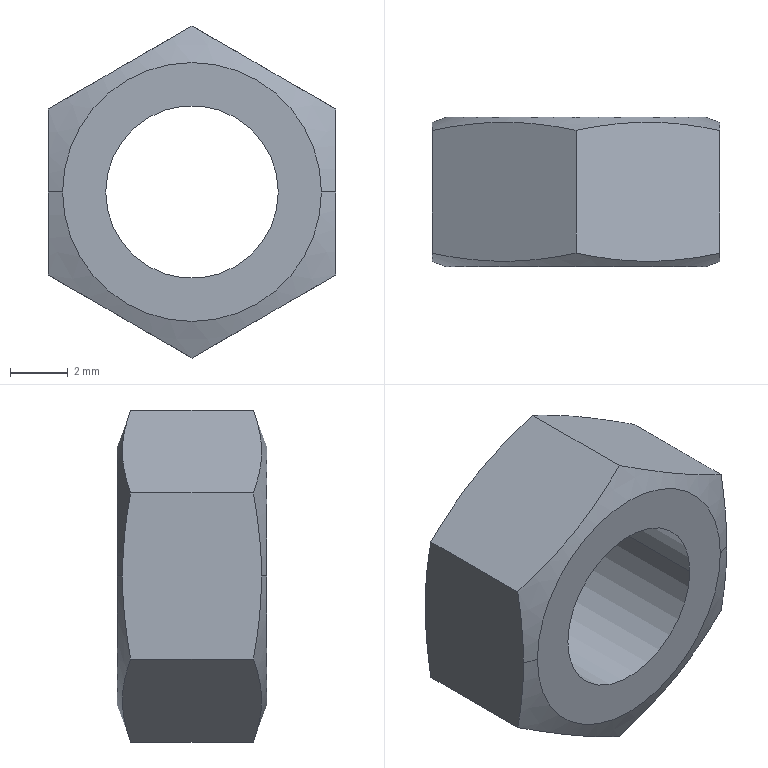Component | SolidWorks | HexNutM6-2 | 1 solid | 14 faces | box 10 x 5.2 x 11.55 mm | volume 296 mm3 | plane 8 | cone 4 | cylinder 2 | commonest cylinder face diameters 6 x2
build123d program:
from build123d import *

# Parameters (mm, degrees)
BOSS_EXTRUDE1_DEPTH = 5.2
SKETCH5_R           = 3
CUT_EXTRUDE1_DEPTH  = 10.24


with BuildPart() as part:
    # Sketch1 → Boss-Extrude1 (new body)
    with BuildSketch(Plane.XY):
        Polygon((0, 5.774), (-5, 2.887), (-5, -2.887), (0, -5.774), (5, -2.887), (5, 2.887), align=None)
    extrude(amount=BOSS_EXTRUDE1_DEPTH)

    # Sketch4 → Cut-Revolve1 (revolve, cut)
    with BuildSketch(Plane(origin=(0, 0, 0), x_dir=(0, 0, -1), z_dir=(1, 0, 0)), mode=Mode.PRIVATE) as cut_revolve1_sk:
        Polygon((-5.2, -4.5), (-4.736, -5.774), (-5.2, -5.774), align=None)
    cut_revolve1 = revolve(cut_revolve1_sk.sketch.rotate(Axis((0, 0, 5.2), (0, 0, -1)), 120), axis=Axis((0, 0, 5.2), (0, 0, -1)), mode=Mode.SUBTRACT)

    # Mirror1: Cut-Revolve1 across plane
    add(cut_revolve1.mirror(Plane.XY.offset(2.6)), mode=Mode.SUBTRACT)

    # Sketch5 → Cut-Extrude1 (cut, through all)
    with BuildSketch(Plane.XY.offset(5.2)):
        Circle(SKETCH5_R)
    extrude(amount=-CUT_EXTRUDE1_DEPTH, mode=Mode.SUBTRACT)


solid = part.part

# Placed as in the assembly
solid = solid.moved(Location((-174.718, -36.4, 23), (90, 0, 0)))
STEP:
#1=CARTESIAN_POINT('',(-6.997,-1.433,0.9055));
#2=VERTEX_POINT('',#1);
#3=CARTESIAN_POINT('',(-6.761,-1.433,0.9055));
#4=VERTEX_POINT('',#3);
#5=CARTESIAN_POINT('',(-6.879,-1.433,0.9055));
#6=DIRECTION('',(0.,-1.,0.));
#7=DIRECTION('',(1.,0.,0.));
#8=AXIS2_PLACEMENT_3D('',#5,#6,#7);
#9=CIRCLE('',#8,0.1181);
#10=EDGE_CURVE('',#2,#4,#9,.T.);
#11=ORIENTED_EDGE('',*,*,#10,.F.);
#12=CARTESIAN_POINT('',(-6.997,-1.638,0.9055));
#13=VERTEX_POINT('',#12);
#14=CARTESIAN_POINT('',(-6.997,-1.433,0.9055));
#15=DIRECTION('',(0.,-1.,0.));
#16=VECTOR('',#15,39.37);
#17=LINE('',#14,#16);
#18=EDGE_CURVE('',#2,#13,#17,.T.);
#19=ORIENTED_EDGE('',*,*,#18,.T.);
#20=CARTESIAN_POINT('',(-6.761,-1.638,0.9055));
#21=VERTEX_POINT('',#20);
#22=CARTESIAN_POINT('',(-6.879,-1.638,0.9055));
#23=DIRECTION('',(0.,-1.,0.));
#24=DIRECTION('',(1.,0.,0.));
#25=AXIS2_PLACEMENT_3D('',#22,#23,#24);
#26=CIRCLE('',#25,0.1181);
#27=EDGE_CURVE('',#13,#21,#26,.T.);
#28=ORIENTED_EDGE('',*,*,#27,.T.);
#29=CARTESIAN_POINT('',(-6.761,-1.433,0.9055));
#30=DIRECTION('',(0.,-1.,0.));
#31=VECTOR('',#30,39.37);
#32=LINE('',#29,#31);
#33=EDGE_CURVE('',#4,#21,#32,.T.);
#34=ORIENTED_EDGE('',*,*,#33,.F.);
#35=EDGE_LOOP('',(#11,#19,#28,#34));
#36=FACE_OUTER_BOUND('',#35,.T.);
#37=CARTESIAN_POINT('',(-6.879,-1.433,0.9055));
#38=DIRECTION('',(0.,-1.,0.));
#39=DIRECTION('',(1.,0.,0.));
#40=AXIS2_PLACEMENT_3D('',#37,#38,#39);
#41=CYLINDRICAL_SURFACE('',#40,0.1181);
#42=ADVANCED_FACE('',(#36),#41,.F.);
#43=CARTESIAN_POINT('',(-7.056,-1.433,0.9055));
#44=VERTEX_POINT('',#43);
#45=CARTESIAN_POINT('',(-6.702,-1.433,0.9055));
#46=VERTEX_POINT('',#45);
#47=CARTESIAN_POINT('',(-6.879,-1.433,0.9055));
#48=DIRECTION('',(0.,-1.,0.));
#49=DIRECTION('',(1.,0.,0.));
#50=AXIS2_PLACEMENT_3D('',#47,#48,#49);
#51=CIRCLE('',#50,0.1772);
#52=EDGE_CURVE('',#44,#46,#51,.T.);
#53=ORIENTED_EDGE('',*,*,#52,.T.);
#54=CARTESIAN_POINT('',(-6.682,-1.44,0.9055));
#55=VERTEX_POINT('',#54);
#56=CARTESIAN_POINT('',(-6.651,-1.451,0.9055));
#57=DIRECTION('',(0.9397,-0.342,-0.));
#58=VECTOR('',#57,39.37);
#59=LINE('',#56,#58);
#60=EDGE_CURVE('',#46,#55,#59,.T.);
#61=ORIENTED_EDGE('',*,*,#60,.T.);
#62=CARTESIAN_POINT('',(-6.682,-1.451,0.7919));
#63=VERTEX_POINT('',#62);
#64=CARTESIAN_POINT('',(-6.682,-1.451,0.7919));
#65=CARTESIAN_POINT('',(-6.682,-1.448,0.8107));
#66=CARTESIAN_POINT('',(-6.682,-1.445,0.8297));
#67=CARTESIAN_POINT('',(-6.682,-1.441,0.8676));
#68=CARTESIAN_POINT('',(-6.682,-1.44,0.8866));
#69=CARTESIAN_POINT('',(-6.682,-1.44,0.9055));
#70=B_SPLINE_CURVE_WITH_KNOTS('',3,(#64,#65,#66,#67,#68,#69),.UNSPECIFIED.,.F.,.F.,(4,2,4),(0.004893,0.006347,0.007802),.UNSPECIFIED.);
#71=EDGE_CURVE('',#63,#55,#70,.T.);
#72=ORIENTED_EDGE('',*,*,#71,.F.);
#73=CARTESIAN_POINT('',(-6.879,-1.451,0.6782));
#74=VERTEX_POINT('',#73);
#75=CARTESIAN_POINT('',(-6.879,-1.451,0.6782));
#76=CARTESIAN_POINT('',(-6.846,-1.444,0.6972));
#77=CARTESIAN_POINT('',(-6.78,-1.436,0.735));
#78=CARTESIAN_POINT('',(-6.715,-1.444,0.7729));
#79=CARTESIAN_POINT('',(-6.682,-1.451,0.7919));
#80=B_SPLINE_CURVE_WITH_KNOTS('',3,(#75,#76,#77,#78,#79),.UNSPECIFIED.,.F.,.F.,(4,1,4),(0.00000023,0.002887,0.005774),.UNSPECIFIED.);
#81=EDGE_CURVE('',#74,#63,#80,.T.);
#82=ORIENTED_EDGE('',*,*,#81,.F.);
#83=CARTESIAN_POINT('',(-7.076,-1.451,0.7919));
#84=VERTEX_POINT('',#83);
#85=CARTESIAN_POINT('',(-7.076,-1.451,0.7919));
#86=CARTESIAN_POINT('',(-7.043,-1.444,0.7729));
#87=CARTESIAN_POINT('',(-6.977,-1.436,0.735));
#88=CARTESIAN_POINT('',(-6.911,-1.444,0.6972));
#89=CARTESIAN_POINT('',(-6.879,-1.451,0.6782));
#90=B_SPLINE_CURVE_WITH_KNOTS('',3,(#85,#86,#87,#88,#89),.UNSPECIFIED.,.F.,.F.,(4,1,4),(0.00000023,0.002887,0.005774),.UNSPECIFIED.);
#91=EDGE_CURVE('',#84,#74,#90,.T.);
#92=ORIENTED_EDGE('',*,*,#91,.F.);
#93=CARTESIAN_POINT('',(-7.076,-1.44,0.9055));
#94=VERTEX_POINT('',#93);
#95=CARTESIAN_POINT('',(-7.076,-1.44,0.9055));
#96=CARTESIAN_POINT('',(-7.076,-1.44,0.8866));
#97=CARTESIAN_POINT('',(-7.076,-1.441,0.8676));
#98=CARTESIAN_POINT('',(-7.076,-1.445,0.8297));
#99=CARTESIAN_POINT('',(-7.076,-1.448,0.8107));
#100=CARTESIAN_POINT('',(-7.076,-1.451,0.7919));
#101=B_SPLINE_CURVE_WITH_KNOTS('',3,(#95,#96,#97,#98,#99,#100),.UNSPECIFIED.,.F.,.F.,(4,2,4),(0.01339,0.01484,0.01629),.UNSPECIFIED.);
#102=EDGE_CURVE('',#94,#84,#101,.T.);
#103=ORIENTED_EDGE('',*,*,#102,.F.);
#104=CARTESIAN_POINT('',(-7.106,-1.451,0.9055));
#105=DIRECTION('',(-0.9397,-0.342,0.));
#106=VECTOR('',#105,39.37);
#107=LINE('',#104,#106);
#108=EDGE_CURVE('',#44,#94,#107,.T.);
#109=ORIENTED_EDGE('',*,*,#108,.F.);
#110=EDGE_LOOP('',(#53,#61,#72,#82,#92,#103,#109));
#111=FACE_OUTER_BOUND('',#110,.T.);
#112=CARTESIAN_POINT('',(-6.879,-1.451,0.9055));
#113=DIRECTION('',(0.,-1.,0.));
#114=DIRECTION('',(-1.,0.,0.));
#115=AXIS2_PLACEMENT_3D('',#112,#113,#114);
#116=CONICAL_SURFACE('',#115,0.2273,1.222);
#117=ADVANCED_FACE('',(#111),#116,.T.);
#118=CARTESIAN_POINT('',(-6.702,-1.638,0.9055));
#119=VERTEX_POINT('',#118);
#120=CARTESIAN_POINT('',(-7.056,-1.638,0.9055));
#121=VERTEX_POINT('',#120);
#122=CARTESIAN_POINT('',(-6.879,-1.638,0.9055));
#123=DIRECTION('',(0.,-1.,0.));
#124=DIRECTION('',(1.,0.,0.));
#125=AXIS2_PLACEMENT_3D('',#122,#123,#124);
#126=CIRCLE('',#125,0.1772);
#127=EDGE_CURVE('',#119,#121,#126,.T.);
#128=ORIENTED_EDGE('',*,*,#127,.F.);
#129=CARTESIAN_POINT('',(-6.682,-1.631,0.9055));
#130=VERTEX_POINT('',#129);
#131=CARTESIAN_POINT('',(-6.651,-1.62,0.9055));
#132=DIRECTION('',(0.9397,0.342,0.));
#133=VECTOR('',#132,39.37);
#134=LINE('',#131,#133);
#135=EDGE_CURVE('',#119,#130,#134,.T.);
#136=ORIENTED_EDGE('',*,*,#135,.T.);
#137=CARTESIAN_POINT('',(-6.682,-1.62,1.019));
#138=VERTEX_POINT('',#137);
#139=CARTESIAN_POINT('',(-6.682,-1.62,1.019));
#140=CARTESIAN_POINT('',(-6.682,-1.626,0.9814));
#141=CARTESIAN_POINT('',(-6.682,-1.631,0.9435));
#142=CARTESIAN_POINT('',(-6.682,-1.631,0.9055));
#143=B_SPLINE_CURVE_WITH_KNOTS('',3,(#139,#140,#141,#142),.UNSPECIFIED.,.F.,.F.,(4,4),(0.01048,0.01339),.UNSPECIFIED.);
#144=EDGE_CURVE('',#138,#130,#143,.T.);
#145=ORIENTED_EDGE('',*,*,#144,.F.);
#146=CARTESIAN_POINT('',(-6.879,-1.62,1.133));
#147=VERTEX_POINT('',#146);
#148=CARTESIAN_POINT('',(-6.879,-1.62,1.133));
#149=CARTESIAN_POINT('',(-6.846,-1.626,1.114));
#150=CARTESIAN_POINT('',(-6.78,-1.635,1.076));
#151=CARTESIAN_POINT('',(-6.715,-1.626,1.038));
#152=CARTESIAN_POINT('',(-6.682,-1.62,1.019));
#153=B_SPLINE_CURVE_WITH_KNOTS('',3,(#148,#149,#150,#151,#152),.UNSPECIFIED.,.F.,.F.,(4,1,4),(0.00000023,0.002887,0.005774),.UNSPECIFIED.);
#154=EDGE_CURVE('',#147,#138,#153,.T.);
#155=ORIENTED_EDGE('',*,*,#154,.F.);
#156=CARTESIAN_POINT('',(-7.076,-1.62,1.019));
#157=VERTEX_POINT('',#156);
#158=CARTESIAN_POINT('',(-7.076,-1.62,1.019));
#159=CARTESIAN_POINT('',(-7.043,-1.626,1.038));
#160=CARTESIAN_POINT('',(-6.977,-1.635,1.076));
#161=CARTESIAN_POINT('',(-6.911,-1.626,1.114));
#162=CARTESIAN_POINT('',(-6.879,-1.62,1.133));
#163=B_SPLINE_CURVE_WITH_KNOTS('',3,(#158,#159,#160,#161,#162),.UNSPECIFIED.,.F.,.F.,(4,1,4),(0.00000023,0.002887,0.005774),.UNSPECIFIED.);
#164=EDGE_CURVE('',#157,#147,#163,.T.);
#165=ORIENTED_EDGE('',*,*,#164,.F.);
#166=CARTESIAN_POINT('',(-7.076,-1.631,0.9055));
#167=VERTEX_POINT('',#166);
#168=CARTESIAN_POINT('',(-7.076,-1.631,0.9055));
#169=CARTESIAN_POINT('',(-7.076,-1.631,0.9435));
#170=CARTESIAN_POINT('',(-7.076,-1.626,0.9814));
#171=CARTESIAN_POINT('',(-7.076,-1.62,1.019));
#172=B_SPLINE_CURVE_WITH_KNOTS('',3,(#168,#169,#170,#171),.UNSPECIFIED.,.F.,.F.,(4,4),(0.007802,0.01072),.UNSPECIFIED.);
#173=EDGE_CURVE('',#167,#157,#172,.T.);
#174=ORIENTED_EDGE('',*,*,#173,.F.);
#175=CARTESIAN_POINT('',(-7.106,-1.62,0.9055));
#176=DIRECTION('',(-0.9397,0.342,0.));
#177=VECTOR('',#176,39.37);
#178=LINE('',#175,#177);
#179=EDGE_CURVE('',#121,#167,#178,.T.);
#180=ORIENTED_EDGE('',*,*,#179,.F.);
#181=EDGE_LOOP('',(#128,#136,#145,#155,#165,#174,#180));
#182=FACE_OUTER_BOUND('',#181,.T.);
#183=CARTESIAN_POINT('',(-6.879,-1.62,0.9055));
#184=DIRECTION('',(0.,1.,0.));
#185=DIRECTION('',(-1.,0.,0.));
#186=AXIS2_PLACEMENT_3D('',#183,#184,#185);
#187=CONICAL_SURFACE('',#186,0.2273,1.222);
#188=ADVANCED_FACE('',(#182),#187,.T.);
#189=CARTESIAN_POINT('',(-6.682,-1.451,1.019));
#190=VERTEX_POINT('',#189);
#191=CARTESIAN_POINT('',(-6.682,-1.638,1.019));
#192=DIRECTION('',(0.,1.,0.));
#193=VECTOR('',#192,39.37);
#194=LINE('',#191,#193);
#195=EDGE_CURVE('',#138,#190,#194,.T.);
#196=ORIENTED_EDGE('',*,*,#195,.T.);
#197=CARTESIAN_POINT('',(-6.879,-1.451,1.133));
#198=VERTEX_POINT('',#197);
#199=CARTESIAN_POINT('',(-6.682,-1.451,1.019));
#200=CARTESIAN_POINT('',(-6.715,-1.444,1.038));
#201=CARTESIAN_POINT('',(-6.78,-1.436,1.076));
#202=CARTESIAN_POINT('',(-6.846,-1.444,1.114));
#203=CARTESIAN_POINT('',(-6.879,-1.451,1.133));
#204=B_SPLINE_CURVE_WITH_KNOTS('',3,(#199,#200,#201,#202,#203),.UNSPECIFIED.,.F.,.F.,(4,1,4),(0.00000023,0.002887,0.005774),.UNSPECIFIED.);
#205=EDGE_CURVE('',#190,#198,#204,.T.);
#206=ORIENTED_EDGE('',*,*,#205,.T.);
#207=CARTESIAN_POINT('',(-6.879,-1.638,1.133));
#208=DIRECTION('',(0.,1.,0.));
#209=VECTOR('',#208,39.37);
#210=LINE('',#207,#209);
#211=EDGE_CURVE('',#147,#198,#210,.T.);
#212=ORIENTED_EDGE('',*,*,#211,.F.);
#213=ORIENTED_EDGE('',*,*,#154,.T.);
#214=EDGE_LOOP('',(#196,#206,#212,#213));
#215=FACE_OUTER_BOUND('',#214,.T.);
#216=CARTESIAN_POINT('',(-6.682,-1.638,1.019));
#217=DIRECTION('',(-0.5,0.,-0.866));
#218=DIRECTION('',(0.866,0.,-0.5));
#219=AXIS2_PLACEMENT_3D('',#216,#217,#218);
#220=PLANE('',#219);
#221=ADVANCED_FACE('',(#215),#220,.F.);
#222=ORIENTED_EDGE('',*,*,#211,.T.);
#223=CARTESIAN_POINT('',(-7.076,-1.451,1.019));
#224=VERTEX_POINT('',#223);
#225=CARTESIAN_POINT('',(-6.879,-1.451,1.133));
#226=CARTESIAN_POINT('',(-6.911,-1.444,1.114));
#227=CARTESIAN_POINT('',(-6.977,-1.436,1.076));
#228=CARTESIAN_POINT('',(-7.043,-1.444,1.038));
#229=CARTESIAN_POINT('',(-7.076,-1.451,1.019));
#230=B_SPLINE_CURVE_WITH_KNOTS('',3,(#225,#226,#227,#228,#229),.UNSPECIFIED.,.F.,.F.,(4,1,4),(0.00000023,0.002887,0.005774),.UNSPECIFIED.);
#231=EDGE_CURVE('',#198,#224,#230,.T.);
#232=ORIENTED_EDGE('',*,*,#231,.T.);
#233=CARTESIAN_POINT('',(-7.076,-1.638,1.019));
#234=DIRECTION('',(0.,1.,0.));
#235=VECTOR('',#234,39.37);
#236=LINE('',#233,#235);
#237=EDGE_CURVE('',#157,#224,#236,.T.);
#238=ORIENTED_EDGE('',*,*,#237,.F.);
#239=ORIENTED_EDGE('',*,*,#164,.T.);
#240=EDGE_LOOP('',(#222,#232,#238,#239));
#241=FACE_OUTER_BOUND('',#240,.T.);
#242=CARTESIAN_POINT('',(-6.879,-1.638,1.133));
#243=DIRECTION('',(0.5,0.,-0.866));
#244=DIRECTION('',(0.866,0.,0.5));
#245=AXIS2_PLACEMENT_3D('',#242,#243,#244);
#246=PLANE('',#245);
#247=ADVANCED_FACE('',(#241),#246,.F.);
#248=ORIENTED_EDGE('',*,*,#237,.T.);
#249=CARTESIAN_POINT('',(-7.076,-1.451,1.019));
#250=CARTESIAN_POINT('',(-7.076,-1.444,0.9814));
#251=CARTESIAN_POINT('',(-7.076,-1.44,0.9435));
#252=CARTESIAN_POINT('',(-7.076,-1.44,0.9055));
#253=B_SPLINE_CURVE_WITH_KNOTS('',3,(#249,#250,#251,#252),.UNSPECIFIED.,.F.,.F.,(4,4),(0.01048,0.01339),.UNSPECIFIED.);
#254=EDGE_CURVE('',#224,#94,#253,.T.);
#255=ORIENTED_EDGE('',*,*,#254,.T.);
#256=ORIENTED_EDGE('',*,*,#102,.T.);
#257=CARTESIAN_POINT('',(-7.076,-1.62,0.7919));
#258=VERTEX_POINT('',#257);
#259=CARTESIAN_POINT('',(-7.076,-1.638,0.7919));
#260=DIRECTION('',(0.,1.,0.));
#261=VECTOR('',#260,39.37);
#262=LINE('',#259,#261);
#263=EDGE_CURVE('',#258,#84,#262,.T.);
#264=ORIENTED_EDGE('',*,*,#263,.F.);
#265=CARTESIAN_POINT('',(-7.076,-1.62,0.7919));
#266=CARTESIAN_POINT('',(-7.076,-1.623,0.8107));
#267=CARTESIAN_POINT('',(-7.076,-1.626,0.8297));
#268=CARTESIAN_POINT('',(-7.076,-1.63,0.8676));
#269=CARTESIAN_POINT('',(-7.076,-1.631,0.8866));
#270=CARTESIAN_POINT('',(-7.076,-1.631,0.9055));
#271=B_SPLINE_CURVE_WITH_KNOTS('',3,(#265,#266,#267,#268,#269,#270),.UNSPECIFIED.,.F.,.F.,(4,2,4),(0.004893,0.006347,0.007802),.UNSPECIFIED.);
#272=EDGE_CURVE('',#258,#167,#271,.T.);
#273=ORIENTED_EDGE('',*,*,#272,.T.);
#274=ORIENTED_EDGE('',*,*,#173,.T.);
#275=EDGE_LOOP('',(#248,#255,#256,#264,#273,#274));
#276=FACE_OUTER_BOUND('',#275,.T.);
#277=CARTESIAN_POINT('',(-7.076,-1.638,1.019));
#278=DIRECTION('',(1.,0.,-0.));
#279=DIRECTION('',(0.,0.,1.));
#280=AXIS2_PLACEMENT_3D('',#277,#278,#279);
#281=PLANE('',#280);
#282=ADVANCED_FACE('',(#276),#281,.F.);
#283=ORIENTED_EDGE('',*,*,#263,.T.);
#284=ORIENTED_EDGE('',*,*,#91,.T.);
#285=CARTESIAN_POINT('',(-6.879,-1.62,0.6782));
#286=VERTEX_POINT('',#285);
#287=CARTESIAN_POINT('',(-6.879,-1.638,0.6782));
#288=DIRECTION('',(0.,1.,0.));
#289=VECTOR('',#288,39.37);
#290=LINE('',#287,#289);
#291=EDGE_CURVE('',#286,#74,#290,.T.);
#292=ORIENTED_EDGE('',*,*,#291,.F.);
#293=CARTESIAN_POINT('',(-6.879,-1.62,0.6782));
#294=CARTESIAN_POINT('',(-6.911,-1.626,0.6972));
#295=CARTESIAN_POINT('',(-6.977,-1.635,0.735));
#296=CARTESIAN_POINT('',(-7.043,-1.626,0.7729));
#297=CARTESIAN_POINT('',(-7.076,-1.62,0.7919));
#298=B_SPLINE_CURVE_WITH_KNOTS('',3,(#293,#294,#295,#296,#297),.UNSPECIFIED.,.F.,.F.,(4,1,4),(0.00000023,0.002887,0.005774),.UNSPECIFIED.);
#299=EDGE_CURVE('',#286,#258,#298,.T.);
#300=ORIENTED_EDGE('',*,*,#299,.T.);
#301=EDGE_LOOP('',(#283,#284,#292,#300));
#302=FACE_OUTER_BOUND('',#301,.T.);
#303=CARTESIAN_POINT('',(-7.076,-1.638,0.7919));
#304=DIRECTION('',(0.5,0.,0.866));
#305=DIRECTION('',(-0.866,0.,0.5));
#306=AXIS2_PLACEMENT_3D('',#303,#304,#305);
#307=PLANE('',#306);
#308=ADVANCED_FACE('',(#302),#307,.F.);
#309=ORIENTED_EDGE('',*,*,#291,.T.);
#310=ORIENTED_EDGE('',*,*,#81,.T.);
#311=CARTESIAN_POINT('',(-6.682,-1.62,0.7919));
#312=VERTEX_POINT('',#311);
#313=CARTESIAN_POINT('',(-6.682,-1.638,0.7919));
#314=DIRECTION('',(0.,1.,0.));
#315=VECTOR('',#314,39.37);
#316=LINE('',#313,#315);
#317=EDGE_CURVE('',#312,#63,#316,.T.);
#318=ORIENTED_EDGE('',*,*,#317,.F.);
#319=CARTESIAN_POINT('',(-6.682,-1.62,0.7919));
#320=CARTESIAN_POINT('',(-6.715,-1.626,0.7729));
#321=CARTESIAN_POINT('',(-6.78,-1.635,0.735));
#322=CARTESIAN_POINT('',(-6.846,-1.626,0.6972));
#323=CARTESIAN_POINT('',(-6.879,-1.62,0.6782));
#324=B_SPLINE_CURVE_WITH_KNOTS('',3,(#319,#320,#321,#322,#323),.UNSPECIFIED.,.F.,.F.,(4,1,4),(0.00000023,0.002887,0.005774),.UNSPECIFIED.);
#325=EDGE_CURVE('',#312,#286,#324,.T.);
#326=ORIENTED_EDGE('',*,*,#325,.T.);
#327=EDGE_LOOP('',(#309,#310,#318,#326));
#328=FACE_OUTER_BOUND('',#327,.T.);
#329=CARTESIAN_POINT('',(-6.879,-1.638,0.6782));
#330=DIRECTION('',(-0.5,0.,0.866));
#331=DIRECTION('',(-0.866,0.,-0.5));
#332=AXIS2_PLACEMENT_3D('',#329,#330,#331);
#333=PLANE('',#332);
#334=ADVANCED_FACE('',(#328),#333,.F.);
#335=ORIENTED_EDGE('',*,*,#317,.T.);
#336=ORIENTED_EDGE('',*,*,#71,.T.);
#337=CARTESIAN_POINT('',(-6.682,-1.44,0.9055));
#338=CARTESIAN_POINT('',(-6.682,-1.44,0.9435));
#339=CARTESIAN_POINT('',(-6.682,-1.444,0.9814));
#340=CARTESIAN_POINT('',(-6.682,-1.451,1.019));
#341=B_SPLINE_CURVE_WITH_KNOTS('',3,(#337,#338,#339,#340),.UNSPECIFIED.,.F.,.F.,(4,4),(0.007802,0.01072),.UNSPECIFIED.);
#342=EDGE_CURVE('',#55,#190,#341,.T.);
#343=ORIENTED_EDGE('',*,*,#342,.T.);
#344=ORIENTED_EDGE('',*,*,#195,.F.);
#345=ORIENTED_EDGE('',*,*,#144,.T.);
#346=CARTESIAN_POINT('',(-6.682,-1.631,0.9055));
#347=CARTESIAN_POINT('',(-6.682,-1.631,0.8866));
#348=CARTESIAN_POINT('',(-6.682,-1.63,0.8676));
#349=CARTESIAN_POINT('',(-6.682,-1.626,0.8297));
#350=CARTESIAN_POINT('',(-6.682,-1.623,0.8107));
#351=CARTESIAN_POINT('',(-6.682,-1.62,0.7919));
#352=B_SPLINE_CURVE_WITH_KNOTS('',3,(#346,#347,#348,#349,#350,#351),.UNSPECIFIED.,.F.,.F.,(4,2,4),(0.01339,0.01484,0.01629),.UNSPECIFIED.);
#353=EDGE_CURVE('',#130,#312,#352,.T.);
#354=ORIENTED_EDGE('',*,*,#353,.T.);
#355=EDGE_LOOP('',(#335,#336,#343,#344,#345,#354));
#356=FACE_OUTER_BOUND('',#355,.T.);
#357=CARTESIAN_POINT('',(-6.682,-1.638,0.7919));
#358=DIRECTION('',(-1.,0.,-0.));
#359=DIRECTION('',(0.,0.,-1.));
#360=AXIS2_PLACEMENT_3D('',#357,#358,#359);
#361=PLANE('',#360);
#362=ADVANCED_FACE('',(#356),#361,.F.);
#363=ORIENTED_EDGE('',*,*,#135,.F.);
#364=CARTESIAN_POINT('',(-6.879,-1.638,0.9055));
#365=DIRECTION('',(0.,-1.,0.));
#366=DIRECTION('',(1.,0.,0.));
#367=AXIS2_PLACEMENT_3D('',#364,#365,#366);
#368=CIRCLE('',#367,0.1772);
#369=EDGE_CURVE('',#121,#119,#368,.T.);
#370=ORIENTED_EDGE('',*,*,#369,.F.);
#371=ORIENTED_EDGE('',*,*,#179,.T.);
#372=ORIENTED_EDGE('',*,*,#272,.F.);
#373=ORIENTED_EDGE('',*,*,#299,.F.);
#374=ORIENTED_EDGE('',*,*,#325,.F.);
#375=ORIENTED_EDGE('',*,*,#353,.F.);
#376=EDGE_LOOP('',(#363,#370,#371,#372,#373,#374,#375));
#377=FACE_OUTER_BOUND('',#376,.T.);
#378=CARTESIAN_POINT('',(-6.879,-1.62,0.9055));
#379=DIRECTION('',(0.,1.,0.));
#380=DIRECTION('',(-1.,0.,0.));
#381=AXIS2_PLACEMENT_3D('',#378,#379,#380);
#382=CONICAL_SURFACE('',#381,0.2273,1.222);
#383=ADVANCED_FACE('',(#377),#382,.T.);
#384=CARTESIAN_POINT('',(-6.879,-1.638,0.9055));
#385=DIRECTION('',(0.,-1.,0.));
#386=DIRECTION('',(1.,0.,0.));
#387=AXIS2_PLACEMENT_3D('',#384,#385,#386);
#388=CIRCLE('',#387,0.1181);
#389=EDGE_CURVE('',#21,#13,#388,.T.);
#390=ORIENTED_EDGE('',*,*,#389,.F.);
#391=ORIENTED_EDGE('',*,*,#27,.F.);
#392=EDGE_LOOP('',(#390,#391));
#393=FACE_BOUND('',#392,.T.);
#394=ORIENTED_EDGE('',*,*,#369,.T.);
#395=ORIENTED_EDGE('',*,*,#127,.T.);
#396=EDGE_LOOP('',(#394,#395));
#397=FACE_OUTER_BOUND('',#396,.T.);
#398=CARTESIAN_POINT('',(-6.879,-1.638,0.9055));
#399=DIRECTION('',(0.,-1.,0.));
#400=DIRECTION('',(1.,0.,0.));
#401=AXIS2_PLACEMENT_3D('',#398,#399,#400);
#402=PLANE('',#401);
#403=ADVANCED_FACE('',(#393,#397),#402,.T.);
#404=ORIENTED_EDGE('',*,*,#60,.F.);
#405=CARTESIAN_POINT('',(-6.879,-1.433,0.9055));
#406=DIRECTION('',(0.,-1.,0.));
#407=DIRECTION('',(1.,0.,0.));
#408=AXIS2_PLACEMENT_3D('',#405,#406,#407);
#409=CIRCLE('',#408,0.1772);
#410=EDGE_CURVE('',#46,#44,#409,.T.);
#411=ORIENTED_EDGE('',*,*,#410,.T.);
#412=ORIENTED_EDGE('',*,*,#108,.T.);
#413=ORIENTED_EDGE('',*,*,#254,.F.);
#414=ORIENTED_EDGE('',*,*,#231,.F.);
#415=ORIENTED_EDGE('',*,*,#205,.F.);
#416=ORIENTED_EDGE('',*,*,#342,.F.);
#417=EDGE_LOOP('',(#404,#411,#412,#413,#414,#415,#416));
#418=FACE_OUTER_BOUND('',#417,.T.);
#419=CARTESIAN_POINT('',(-6.879,-1.451,0.9055));
#420=DIRECTION('',(0.,-1.,0.));
#421=DIRECTION('',(-1.,0.,0.));
#422=AXIS2_PLACEMENT_3D('',#419,#420,#421);
#423=CONICAL_SURFACE('',#422,0.2273,1.222);
#424=ADVANCED_FACE('',(#418),#423,.T.);
#425=CARTESIAN_POINT('',(-6.879,-1.433,0.9055));
#426=DIRECTION('',(0.,-1.,0.));
#427=DIRECTION('',(1.,0.,0.));
#428=AXIS2_PLACEMENT_3D('',#425,#426,#427);
#429=CIRCLE('',#428,0.1181);
#430=EDGE_CURVE('',#4,#2,#429,.T.);
#431=ORIENTED_EDGE('',*,*,#430,.T.);
#432=ORIENTED_EDGE('',*,*,#10,.T.);
#433=EDGE_LOOP('',(#431,#432));
#434=FACE_BOUND('',#433,.T.);
#435=ORIENTED_EDGE('',*,*,#52,.F.);
#436=ORIENTED_EDGE('',*,*,#410,.F.);
#437=EDGE_LOOP('',(#435,#436));
#438=FACE_OUTER_BOUND('',#437,.T.);
#439=CARTESIAN_POINT('',(-6.879,-1.433,0.9055));
#440=DIRECTION('',(0.,-1.,0.));
#441=DIRECTION('',(1.,0.,0.));
#442=AXIS2_PLACEMENT_3D('',#439,#440,#441);
#443=PLANE('',#442);
#444=ADVANCED_FACE('',(#434,#438),#443,.F.);
#445=ORIENTED_EDGE('',*,*,#18,.F.);
#446=ORIENTED_EDGE('',*,*,#430,.F.);
#447=ORIENTED_EDGE('',*,*,#33,.T.);
#448=ORIENTED_EDGE('',*,*,#389,.T.);
#449=EDGE_LOOP('',(#445,#446,#447,#448));
#450=FACE_OUTER_BOUND('',#449,.T.);
#451=CARTESIAN_POINT('',(-6.879,-1.433,0.9055));
#452=DIRECTION('',(0.,-1.,0.));
#453=DIRECTION('',(1.,0.,0.));
#454=AXIS2_PLACEMENT_3D('',#451,#452,#453);
#455=CYLINDRICAL_SURFACE('',#454,0.1181);
#456=ADVANCED_FACE('',(#450),#455,.F.);
#457=CLOSED_SHELL('',(#42,#117,#188,#221,#247,#282,#308,#334,#362,#383,#403,#424,#444,#456));
#458=MANIFOLD_SOLID_BREP('',#457);
#459=CARTESIAN_POINT('',(0.,0.,0.));
#460=DIRECTION('',(0.,0.,1.));
#461=DIRECTION('',(1.,0.,0.));
#462=AXIS2_PLACEMENT_3D('',#459,#460,#461);
#463=(LENGTH_UNIT()NAMED_UNIT(*)SI_UNIT($,.METRE.));
#464=LENGTH_MEASURE_WITH_UNIT(LENGTH_MEASURE(0.0254),#463);
#465=DIMENSIONAL_EXPONENTS(1.,0.,0.,0.,0.,0.,0.);
#466=(CONVERSION_BASED_UNIT('',#464)LENGTH_UNIT()NAMED_UNIT(#465));
#467=UNCERTAINTY_MEASURE_WITH_UNIT(LENGTH_MEASURE(0.00001),#466,'','');
#468=(NAMED_UNIT(*)PLANE_ANGLE_UNIT()SI_UNIT($,.RADIAN.));
#469=(NAMED_UNIT(*)SI_UNIT($,.STERADIAN.)SOLID_ANGLE_UNIT());
#470=(GEOMETRIC_REPRESENTATION_CONTEXT(3)GLOBAL_UNCERTAINTY_ASSIGNED_CONTEXT((#467))GLOBAL_UNIT_ASSIGNED_CONTEXT((#466,#468,#469))REPRESENTATION_CONTEXT('',''));
#471=ADVANCED_BREP_SHAPE_REPRESENTATION('',(#458,#462),#470);
#472=COLOUR_RGB('',0.7922,0.8196,0.9333);
#473=FILL_AREA_STYLE_COLOUR('',#472);
#474=FILL_AREA_STYLE('',(#473));
#475=SURFACE_STYLE_FILL_AREA(#474);
#476=SURFACE_SIDE_STYLE('',(#475));
#477=SURFACE_STYLE_USAGE(.BOTH.,#476);
#478=PRESENTATION_STYLE_ASSIGNMENT((#477));
#479=STYLED_ITEM('',(#478),#458);
#480=PRESENTATION_LAYER_ASSIGNMENT('','',(#479));
#481=(LENGTH_UNIT()NAMED_UNIT(*)SI_UNIT($,.METRE.));
#482=LENGTH_MEASURE_WITH_UNIT(LENGTH_MEASURE(0.0254),#481);
#483=DIMENSIONAL_EXPONENTS(1.,0.,0.,0.,0.,0.,0.);
#484=(CONVERSION_BASED_UNIT('',#482)LENGTH_UNIT()NAMED_UNIT(#483));
#485=UNCERTAINTY_MEASURE_WITH_UNIT(LENGTH_MEASURE(0.00001),#484,'','');
#486=(NAMED_UNIT(*)PLANE_ANGLE_UNIT()SI_UNIT($,.RADIAN.));
#487=(NAMED_UNIT(*)SI_UNIT($,.STERADIAN.)SOLID_ANGLE_UNIT());
#488=(GEOMETRIC_REPRESENTATION_CONTEXT(3)GLOBAL_UNCERTAINTY_ASSIGNED_CONTEXT((#485))GLOBAL_UNIT_ASSIGNED_CONTEXT((#484,#486,#487))REPRESENTATION_CONTEXT('',''));
#489=MECHANICAL_DESIGN_GEOMETRIC_PRESENTATION_REPRESENTATION('',(#479),#488);